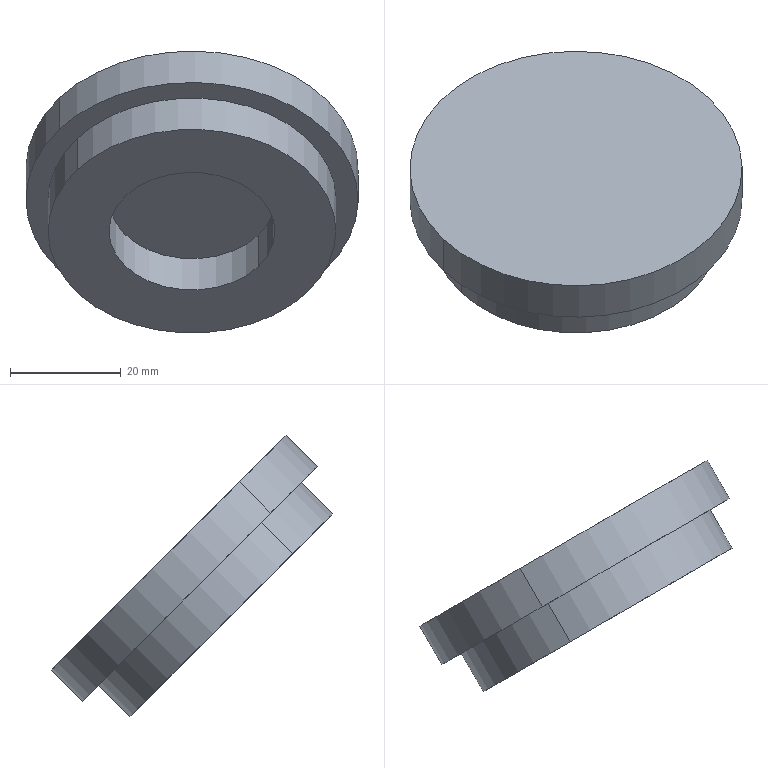Component | SolidWorks | PassiveRollerAssembly-1_NylonCover-1 | 1 solid | 10 faces | box 60 x 50.91 x 50.91 mm | volume 33954 mm3 | cylinder 6 | plane 4 | commonest cylinder face diameters 30 x2 52 x2 60 x2 | material A-Glass Fiber
build123d program:
from build123d import *


with BuildPart() as part:
    # Sketch1 → Revolve1 (revolve)
    with BuildSketch(Plane.XY, mode=Mode.PRIVATE) as revolve1_sk:
        Polygon((0, 0), (0, 30), (8, 30), (8, 26), (16, 26), (16, 15), (8, 15), (8, 0), align=None)
    revolve(revolve1_sk.sketch.rotate(Axis((0, 0, 0), (1, 0, 0)), 90), axis=Axis((0, 0, 0), (1, 0, 0)))


solid = part.part

# Placed as in the assembly
solid = solid.moved(Location((2216.026, 764.545, 398.158), (-135, -84.203, 90)))
STEP:
#1=CARTESIAN_POINT('',(86.774,29.403,15.482));
#2=VERTEX_POINT('',#1);
#3=CARTESIAN_POINT('',(87.716,29.907,14.978));
#4=VERTEX_POINT('',#3);
#5=CARTESIAN_POINT('',(87.245,29.655,15.23));
#6=DIRECTION('',(-0.,0.7071,0.7071));
#7=DIRECTION('',(0.7972,0.4269,-0.4269));
#8=AXIS2_PLACEMENT_3D('',#5,#6,#7);
#9=CIRCLE('',#8,0.5906);
#10=EDGE_CURVE('',#2,#4,#9,.T.);
#11=ORIENTED_EDGE('',*,*,#10,.F.);
#12=CARTESIAN_POINT('',(86.774,29.625,15.705));
#13=VERTEX_POINT('',#12);
#14=CARTESIAN_POINT('',(86.774,29.848,15.928));
#15=DIRECTION('',(-0.,0.7071,0.7071));
#16=VECTOR('',#15,39.37);
#17=LINE('',#14,#16);
#18=EDGE_CURVE('',#2,#13,#17,.T.);
#19=ORIENTED_EDGE('',*,*,#18,.T.);
#20=CARTESIAN_POINT('',(87.716,30.13,15.201));
#21=VERTEX_POINT('',#20);
#22=CARTESIAN_POINT('',(87.245,29.877,15.453));
#23=DIRECTION('',(-0.,0.7071,0.7071));
#24=DIRECTION('',(0.7972,0.4269,-0.4269));
#25=AXIS2_PLACEMENT_3D('',#22,#23,#24);
#26=CIRCLE('',#25,0.5906);
#27=EDGE_CURVE('',#13,#21,#26,.T.);
#28=ORIENTED_EDGE('',*,*,#27,.T.);
#29=CARTESIAN_POINT('',(87.716,30.352,15.423));
#30=DIRECTION('',(-0.,0.7071,0.7071));
#31=VECTOR('',#30,39.37);
#32=LINE('',#29,#31);
#33=EDGE_CURVE('',#4,#21,#32,.T.);
#34=ORIENTED_EDGE('',*,*,#33,.F.);
#35=EDGE_LOOP('',(#11,#19,#28,#34));
#36=FACE_OUTER_BOUND('',#35,.T.);
#37=CARTESIAN_POINT('',(87.245,30.1,15.676));
#38=DIRECTION('',(-0.,0.7071,0.7071));
#39=DIRECTION('',(0.7972,0.4269,-0.4269));
#40=AXIS2_PLACEMENT_3D('',#37,#38,#39);
#41=CYLINDRICAL_SURFACE('',#40,0.5906);
#42=ADVANCED_FACE('',(#36),#41,.F.);
#43=CARTESIAN_POINT('',(88.061,30.092,14.793));
#44=VERTEX_POINT('',#43);
#45=CARTESIAN_POINT('',(86.429,29.218,15.667));
#46=VERTEX_POINT('',#45);
#47=CARTESIAN_POINT('',(87.245,29.655,15.23));
#48=DIRECTION('',(-0.,0.7071,0.7071));
#49=DIRECTION('',(0.7972,0.4269,-0.4269));
#50=AXIS2_PLACEMENT_3D('',#47,#48,#49);
#51=CIRCLE('',#50,1.024);
#52=EDGE_CURVE('',#44,#46,#51,.T.);
#53=ORIENTED_EDGE('',*,*,#52,.T.);
#54=CARTESIAN_POINT('',(86.429,29.44,15.89));
#55=VERTEX_POINT('',#54);
#56=CARTESIAN_POINT('',(86.429,29.663,16.113));
#57=DIRECTION('',(-0.,0.7071,0.7071));
#58=VECTOR('',#57,39.37);
#59=LINE('',#56,#58);
#60=EDGE_CURVE('',#46,#55,#59,.T.);
#61=ORIENTED_EDGE('',*,*,#60,.T.);
#62=CARTESIAN_POINT('',(88.061,30.314,15.016));
#63=VERTEX_POINT('',#62);
#64=CARTESIAN_POINT('',(87.245,29.877,15.453));
#65=DIRECTION('',(-0.,0.7071,0.7071));
#66=DIRECTION('',(0.7972,0.4269,-0.4269));
#67=AXIS2_PLACEMENT_3D('',#64,#65,#66);
#68=CIRCLE('',#67,1.024);
#69=EDGE_CURVE('',#63,#55,#68,.T.);
#70=ORIENTED_EDGE('',*,*,#69,.F.);
#71=CARTESIAN_POINT('',(88.061,30.537,15.239));
#72=DIRECTION('',(-0.,0.7071,0.7071));
#73=VECTOR('',#72,39.37);
#74=LINE('',#71,#73);
#75=EDGE_CURVE('',#44,#63,#74,.T.);
#76=ORIENTED_EDGE('',*,*,#75,.F.);
#77=EDGE_LOOP('',(#53,#61,#70,#76));
#78=FACE_OUTER_BOUND('',#77,.T.);
#79=CARTESIAN_POINT('',(87.245,30.1,15.676));
#80=DIRECTION('',(-0.,0.7071,0.7071));
#81=DIRECTION('',(0.7972,0.4269,-0.4269));
#82=AXIS2_PLACEMENT_3D('',#79,#80,#81);
#83=CYLINDRICAL_SURFACE('',#82,1.024);
#84=ADVANCED_FACE('',(#78),#83,.T.);
#85=CARTESIAN_POINT('',(88.187,30.382,14.949));
#86=VERTEX_POINT('',#85);
#87=CARTESIAN_POINT('',(86.304,29.373,15.957));
#88=VERTEX_POINT('',#87);
#89=CARTESIAN_POINT('',(87.245,29.877,15.453));
#90=DIRECTION('',(-0.,0.7071,0.7071));
#91=DIRECTION('',(0.7972,0.4269,-0.4269));
#92=AXIS2_PLACEMENT_3D('',#89,#90,#91);
#93=CIRCLE('',#92,1.181);
#94=EDGE_CURVE('',#86,#88,#93,.T.);
#95=ORIENTED_EDGE('',*,*,#94,.T.);
#96=CARTESIAN_POINT('',(86.304,29.596,16.18));
#97=VERTEX_POINT('',#96);
#98=CARTESIAN_POINT('',(86.304,29.596,16.18));
#99=DIRECTION('',(-0.,0.7071,0.7071));
#100=VECTOR('',#99,39.37);
#101=LINE('',#98,#100);
#102=EDGE_CURVE('',#88,#97,#101,.T.);
#103=ORIENTED_EDGE('',*,*,#102,.T.);
#104=CARTESIAN_POINT('',(88.187,30.604,15.171));
#105=VERTEX_POINT('',#104);
#106=CARTESIAN_POINT('',(87.245,30.1,15.676));
#107=DIRECTION('',(-0.,0.7071,0.7071));
#108=DIRECTION('',(0.7972,0.4269,-0.4269));
#109=AXIS2_PLACEMENT_3D('',#106,#107,#108);
#110=CIRCLE('',#109,1.181);
#111=EDGE_CURVE('',#105,#97,#110,.T.);
#112=ORIENTED_EDGE('',*,*,#111,.F.);
#113=CARTESIAN_POINT('',(88.187,30.604,15.171));
#114=DIRECTION('',(-0.,0.7071,0.7071));
#115=VECTOR('',#114,39.37);
#116=LINE('',#113,#115);
#117=EDGE_CURVE('',#86,#105,#116,.T.);
#118=ORIENTED_EDGE('',*,*,#117,.F.);
#119=EDGE_LOOP('',(#95,#103,#112,#118));
#120=FACE_OUTER_BOUND('',#119,.T.);
#121=CARTESIAN_POINT('',(87.245,30.1,15.676));
#122=DIRECTION('',(-0.,0.7071,0.7071));
#123=DIRECTION('',(0.7972,0.4269,-0.4269));
#124=AXIS2_PLACEMENT_3D('',#121,#122,#123);
#125=CYLINDRICAL_SURFACE('',#124,1.181);
#126=ADVANCED_FACE('',(#120),#125,.T.);
#127=ORIENTED_EDGE('',*,*,#111,.T.);
#128=CARTESIAN_POINT('',(87.245,30.1,15.676));
#129=DIRECTION('',(-0.,0.7071,0.7071));
#130=DIRECTION('',(0.7972,0.4269,-0.4269));
#131=AXIS2_PLACEMENT_3D('',#128,#129,#130);
#132=CIRCLE('',#131,1.181);
#133=EDGE_CURVE('',#97,#105,#132,.T.);
#134=ORIENTED_EDGE('',*,*,#133,.T.);
#135=EDGE_LOOP('',(#127,#134));
#136=FACE_OUTER_BOUND('',#135,.T.);
#137=CARTESIAN_POINT('',(87.245,30.1,15.676));
#138=DIRECTION('',(0.,-0.7071,-0.7071));
#139=DIRECTION('',(-0.7972,-0.4269,0.4269));
#140=AXIS2_PLACEMENT_3D('',#137,#138,#139);
#141=PLANE('',#140);
#142=ADVANCED_FACE('',(#136),#141,.F.);
#143=ORIENTED_EDGE('',*,*,#102,.F.);
#144=CARTESIAN_POINT('',(87.245,29.877,15.453));
#145=DIRECTION('',(-0.,0.7071,0.7071));
#146=DIRECTION('',(0.7972,0.4269,-0.4269));
#147=AXIS2_PLACEMENT_3D('',#144,#145,#146);
#148=CIRCLE('',#147,1.181);
#149=EDGE_CURVE('',#88,#86,#148,.T.);
#150=ORIENTED_EDGE('',*,*,#149,.T.);
#151=ORIENTED_EDGE('',*,*,#117,.T.);
#152=ORIENTED_EDGE('',*,*,#133,.F.);
#153=EDGE_LOOP('',(#143,#150,#151,#152));
#154=FACE_OUTER_BOUND('',#153,.T.);
#155=CARTESIAN_POINT('',(87.245,30.1,15.676));
#156=DIRECTION('',(-0.,0.7071,0.7071));
#157=DIRECTION('',(0.7972,0.4269,-0.4269));
#158=AXIS2_PLACEMENT_3D('',#155,#156,#157);
#159=CYLINDRICAL_SURFACE('',#158,1.181);
#160=ADVANCED_FACE('',(#154),#159,.T.);
#161=ORIENTED_EDGE('',*,*,#94,.F.);
#162=ORIENTED_EDGE('',*,*,#149,.F.);
#163=EDGE_LOOP('',(#161,#162));
#164=FACE_OUTER_BOUND('',#163,.T.);
#165=ORIENTED_EDGE('',*,*,#69,.T.);
#166=CARTESIAN_POINT('',(87.245,29.877,15.453));
#167=DIRECTION('',(-0.,0.7071,0.7071));
#168=DIRECTION('',(0.7972,0.4269,-0.4269));
#169=AXIS2_PLACEMENT_3D('',#166,#167,#168);
#170=CIRCLE('',#169,1.024);
#171=EDGE_CURVE('',#55,#63,#170,.T.);
#172=ORIENTED_EDGE('',*,*,#171,.T.);
#173=EDGE_LOOP('',(#165,#172));
#174=FACE_BOUND('',#173,.T.);
#175=CARTESIAN_POINT('',(86.532,30.543,14.787));
#176=DIRECTION('',(-0.,0.7071,0.7071));
#177=DIRECTION('',(0.7972,0.4269,-0.4269));
#178=AXIS2_PLACEMENT_3D('',#175,#176,#177);
#179=PLANE('',#178);
#180=ADVANCED_FACE('',(#164,#174),#179,.F.);
#181=ORIENTED_EDGE('',*,*,#60,.F.);
#182=CARTESIAN_POINT('',(87.245,29.655,15.23));
#183=DIRECTION('',(-0.,0.7071,0.7071));
#184=DIRECTION('',(0.7972,0.4269,-0.4269));
#185=AXIS2_PLACEMENT_3D('',#182,#183,#184);
#186=CIRCLE('',#185,1.024);
#187=EDGE_CURVE('',#46,#44,#186,.T.);
#188=ORIENTED_EDGE('',*,*,#187,.T.);
#189=ORIENTED_EDGE('',*,*,#75,.T.);
#190=ORIENTED_EDGE('',*,*,#171,.F.);
#191=EDGE_LOOP('',(#181,#188,#189,#190));
#192=FACE_OUTER_BOUND('',#191,.T.);
#193=CARTESIAN_POINT('',(87.245,30.1,15.676));
#194=DIRECTION('',(-0.,0.7071,0.7071));
#195=DIRECTION('',(0.7972,0.4269,-0.4269));
#196=AXIS2_PLACEMENT_3D('',#193,#194,#195);
#197=CYLINDRICAL_SURFACE('',#196,1.024);
#198=ADVANCED_FACE('',(#192),#197,.T.);
#199=ORIENTED_EDGE('',*,*,#52,.F.);
#200=ORIENTED_EDGE('',*,*,#187,.F.);
#201=EDGE_LOOP('',(#199,#200));
#202=FACE_OUTER_BOUND('',#201,.T.);
#203=CARTESIAN_POINT('',(87.245,29.655,15.23));
#204=DIRECTION('',(-0.,0.7071,0.7071));
#205=DIRECTION('',(0.7972,0.4269,-0.4269));
#206=AXIS2_PLACEMENT_3D('',#203,#204,#205);
#207=CIRCLE('',#206,0.5906);
#208=EDGE_CURVE('',#4,#2,#207,.T.);
#209=ORIENTED_EDGE('',*,*,#208,.T.);
#210=ORIENTED_EDGE('',*,*,#10,.T.);
#211=EDGE_LOOP('',(#209,#210));
#212=FACE_BOUND('',#211,.T.);
#213=CARTESIAN_POINT('',(86.627,30.232,14.653));
#214=DIRECTION('',(-0.,0.7071,0.7071));
#215=DIRECTION('',(0.7972,0.4269,-0.4269));
#216=AXIS2_PLACEMENT_3D('',#213,#214,#215);
#217=PLANE('',#216);
#218=ADVANCED_FACE('',(#202,#212),#217,.F.);
#219=ORIENTED_EDGE('',*,*,#18,.F.);
#220=ORIENTED_EDGE('',*,*,#208,.F.);
#221=ORIENTED_EDGE('',*,*,#33,.T.);
#222=CARTESIAN_POINT('',(87.245,29.877,15.453));
#223=DIRECTION('',(-0.,0.7071,0.7071));
#224=DIRECTION('',(0.7972,0.4269,-0.4269));
#225=AXIS2_PLACEMENT_3D('',#222,#223,#224);
#226=CIRCLE('',#225,0.5906);
#227=EDGE_CURVE('',#21,#13,#226,.T.);
#228=ORIENTED_EDGE('',*,*,#227,.T.);
#229=EDGE_LOOP('',(#219,#220,#221,#228));
#230=FACE_OUTER_BOUND('',#229,.T.);
#231=CARTESIAN_POINT('',(87.245,30.1,15.676));
#232=DIRECTION('',(-0.,0.7071,0.7071));
#233=DIRECTION('',(0.7972,0.4269,-0.4269));
#234=AXIS2_PLACEMENT_3D('',#231,#232,#233);
#235=CYLINDRICAL_SURFACE('',#234,0.5906);
#236=ADVANCED_FACE('',(#230),#235,.F.);
#237=ORIENTED_EDGE('',*,*,#227,.F.);
#238=ORIENTED_EDGE('',*,*,#27,.F.);
#239=EDGE_LOOP('',(#237,#238));
#240=FACE_OUTER_BOUND('',#239,.T.);
#241=CARTESIAN_POINT('',(86.889,30.21,15.12));
#242=DIRECTION('',(-0.,0.7071,0.7071));
#243=DIRECTION('',(0.7972,0.4269,-0.4269));
#244=AXIS2_PLACEMENT_3D('',#241,#242,#243);
#245=PLANE('',#244);
#246=ADVANCED_FACE('',(#240),#245,.F.);
#247=CLOSED_SHELL('',(#42,#84,#126,#142,#160,#180,#198,#218,#236,#246));
#248=MANIFOLD_SOLID_BREP('',#247);
#249=CARTESIAN_POINT('',(0.,0.,0.));
#250=DIRECTION('',(0.,0.,1.));
#251=DIRECTION('',(1.,0.,0.));
#252=AXIS2_PLACEMENT_3D('',#249,#250,#251);
#253=(LENGTH_UNIT()NAMED_UNIT(*)SI_UNIT($,.METRE.));
#254=LENGTH_MEASURE_WITH_UNIT(LENGTH_MEASURE(0.0254),#253);
#255=DIMENSIONAL_EXPONENTS(1.,0.,0.,0.,0.,0.,0.);
#256=(CONVERSION_BASED_UNIT('',#254)LENGTH_UNIT()NAMED_UNIT(#255));
#257=UNCERTAINTY_MEASURE_WITH_UNIT(LENGTH_MEASURE(0.00001),#256,'','');
#258=(NAMED_UNIT(*)PLANE_ANGLE_UNIT()SI_UNIT($,.RADIAN.));
#259=(NAMED_UNIT(*)SI_UNIT($,.STERADIAN.)SOLID_ANGLE_UNIT());
#260=(GEOMETRIC_REPRESENTATION_CONTEXT(3)GLOBAL_UNCERTAINTY_ASSIGNED_CONTEXT((#257))GLOBAL_UNIT_ASSIGNED_CONTEXT((#256,#258,#259))REPRESENTATION_CONTEXT('',''));
#261=ADVANCED_BREP_SHAPE_REPRESENTATION('',(#248,#252),#260);
#262=COLOUR_RGB('',0.7922,0.8196,0.9333);
#263=FILL_AREA_STYLE_COLOUR('',#262);
#264=FILL_AREA_STYLE('',(#263));
#265=SURFACE_STYLE_FILL_AREA(#264);
#266=SURFACE_SIDE_STYLE('',(#265));
#267=SURFACE_STYLE_USAGE(.BOTH.,#266);
#268=PRESENTATION_STYLE_ASSIGNMENT((#267));
#269=STYLED_ITEM('',(#268),#248);
#270=PRESENTATION_LAYER_ASSIGNMENT('','',(#269));
#271=(LENGTH_UNIT()NAMED_UNIT(*)SI_UNIT($,.METRE.));
#272=LENGTH_MEASURE_WITH_UNIT(LENGTH_MEASURE(0.0254),#271);
#273=DIMENSIONAL_EXPONENTS(1.,0.,0.,0.,0.,0.,0.);
#274=(CONVERSION_BASED_UNIT('',#272)LENGTH_UNIT()NAMED_UNIT(#273));
#275=UNCERTAINTY_MEASURE_WITH_UNIT(LENGTH_MEASURE(0.00001),#274,'','');
#276=(NAMED_UNIT(*)PLANE_ANGLE_UNIT()SI_UNIT($,.RADIAN.));
#277=(NAMED_UNIT(*)SI_UNIT($,.STERADIAN.)SOLID_ANGLE_UNIT());
#278=(GEOMETRIC_REPRESENTATION_CONTEXT(3)GLOBAL_UNCERTAINTY_ASSIGNED_CONTEXT((#275))GLOBAL_UNIT_ASSIGNED_CONTEXT((#274,#276,#277))REPRESENTATION_CONTEXT('',''));
#279=MECHANICAL_DESIGN_GEOMETRIC_PRESENTATION_REPRESENTATION('',(#269),#278);